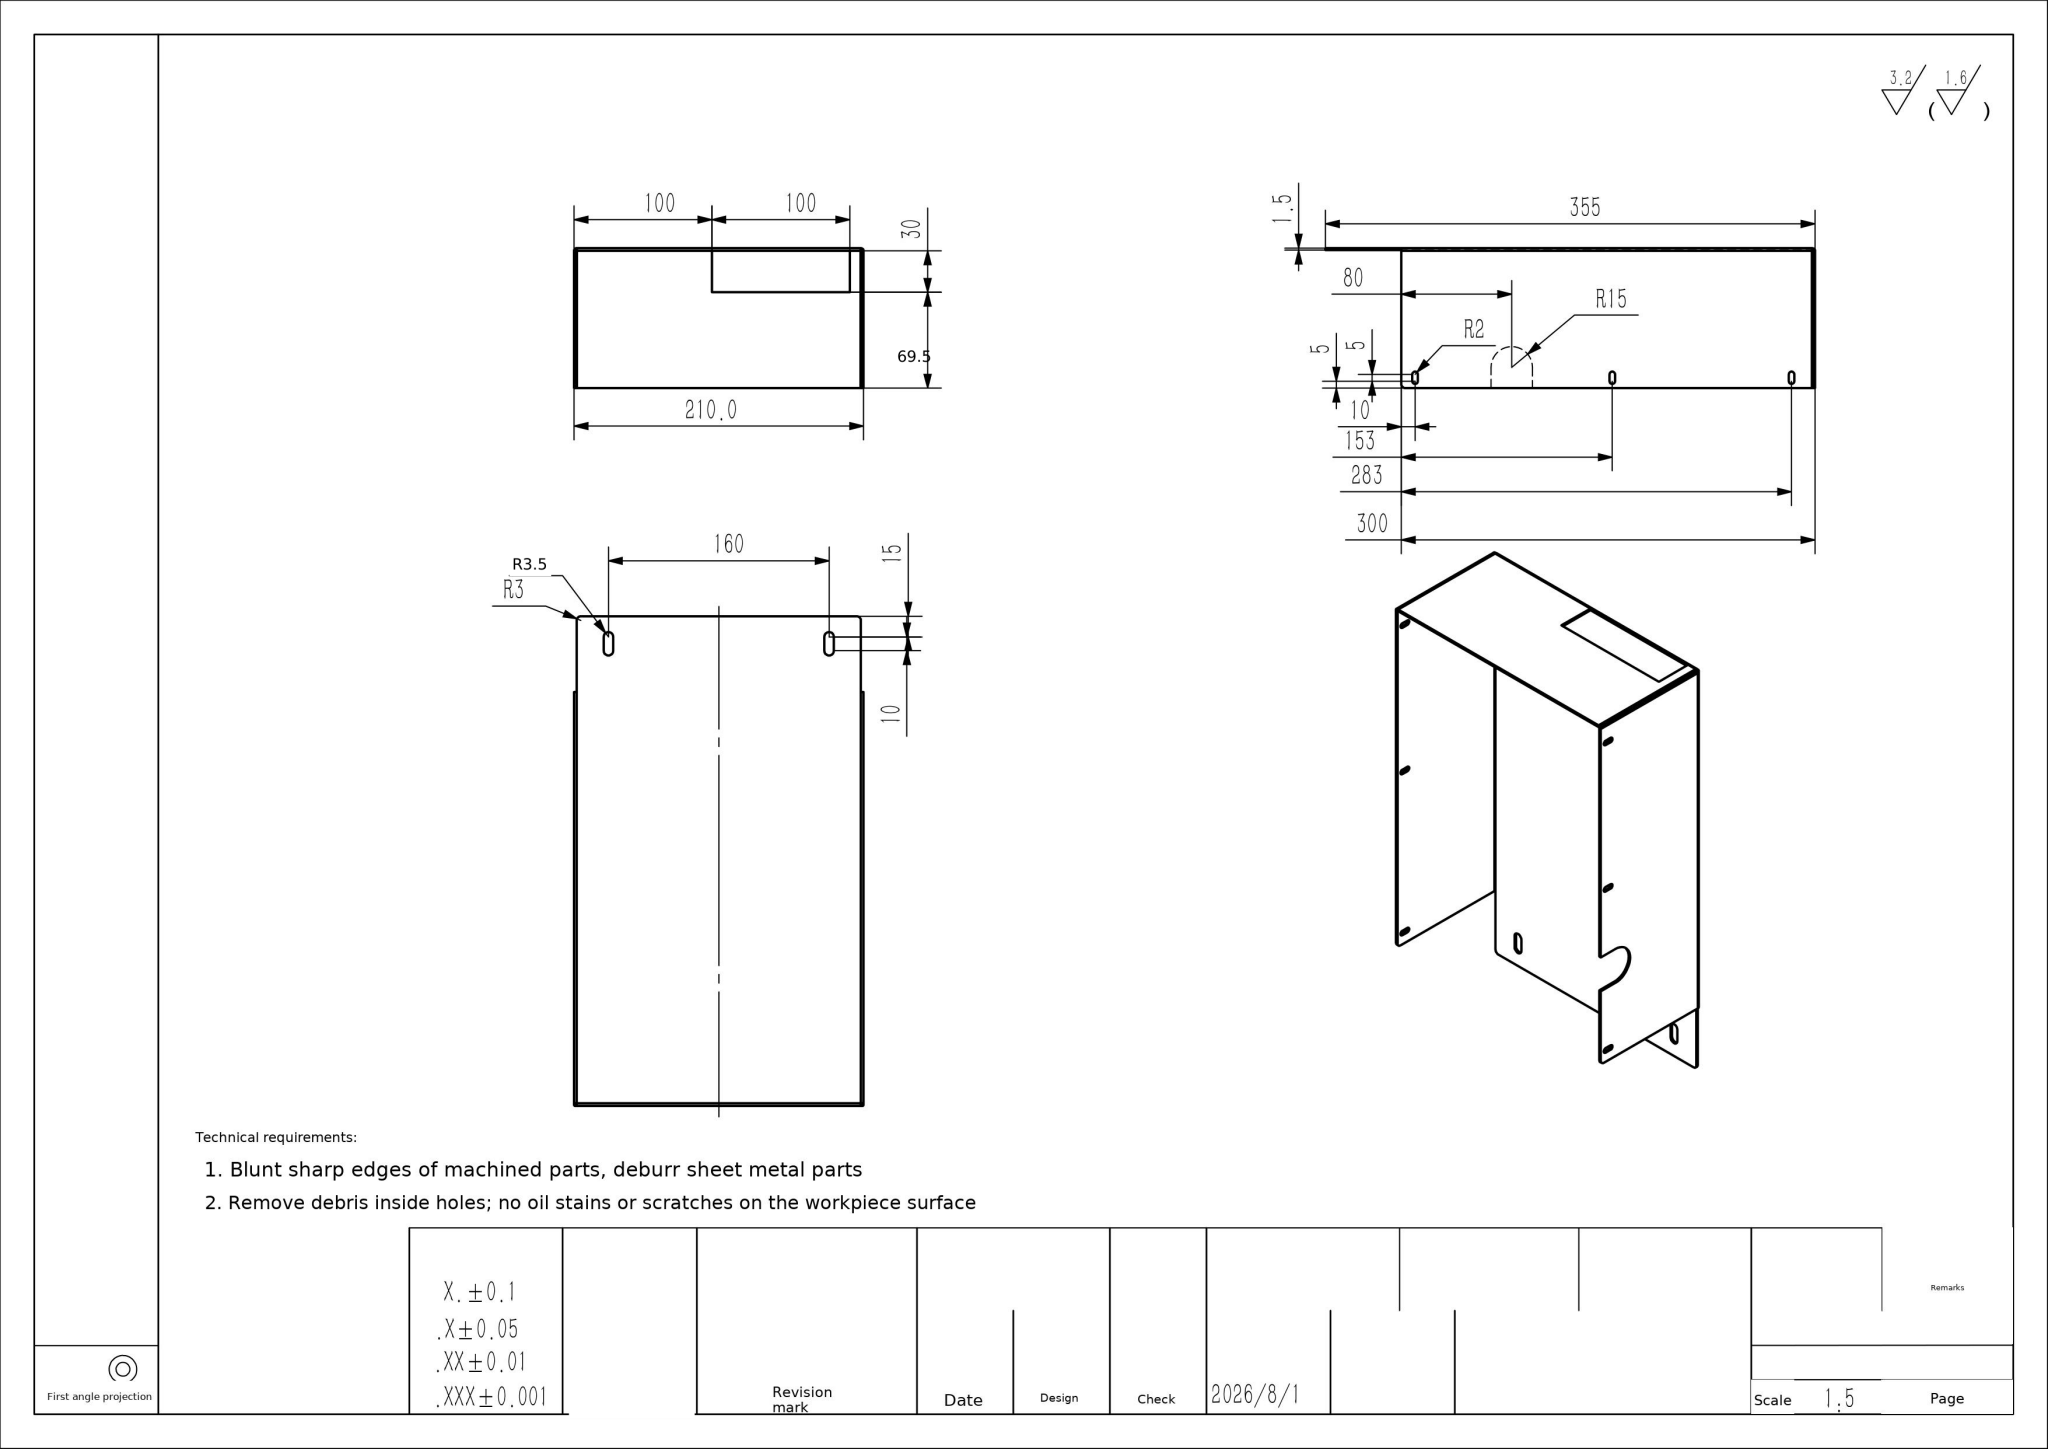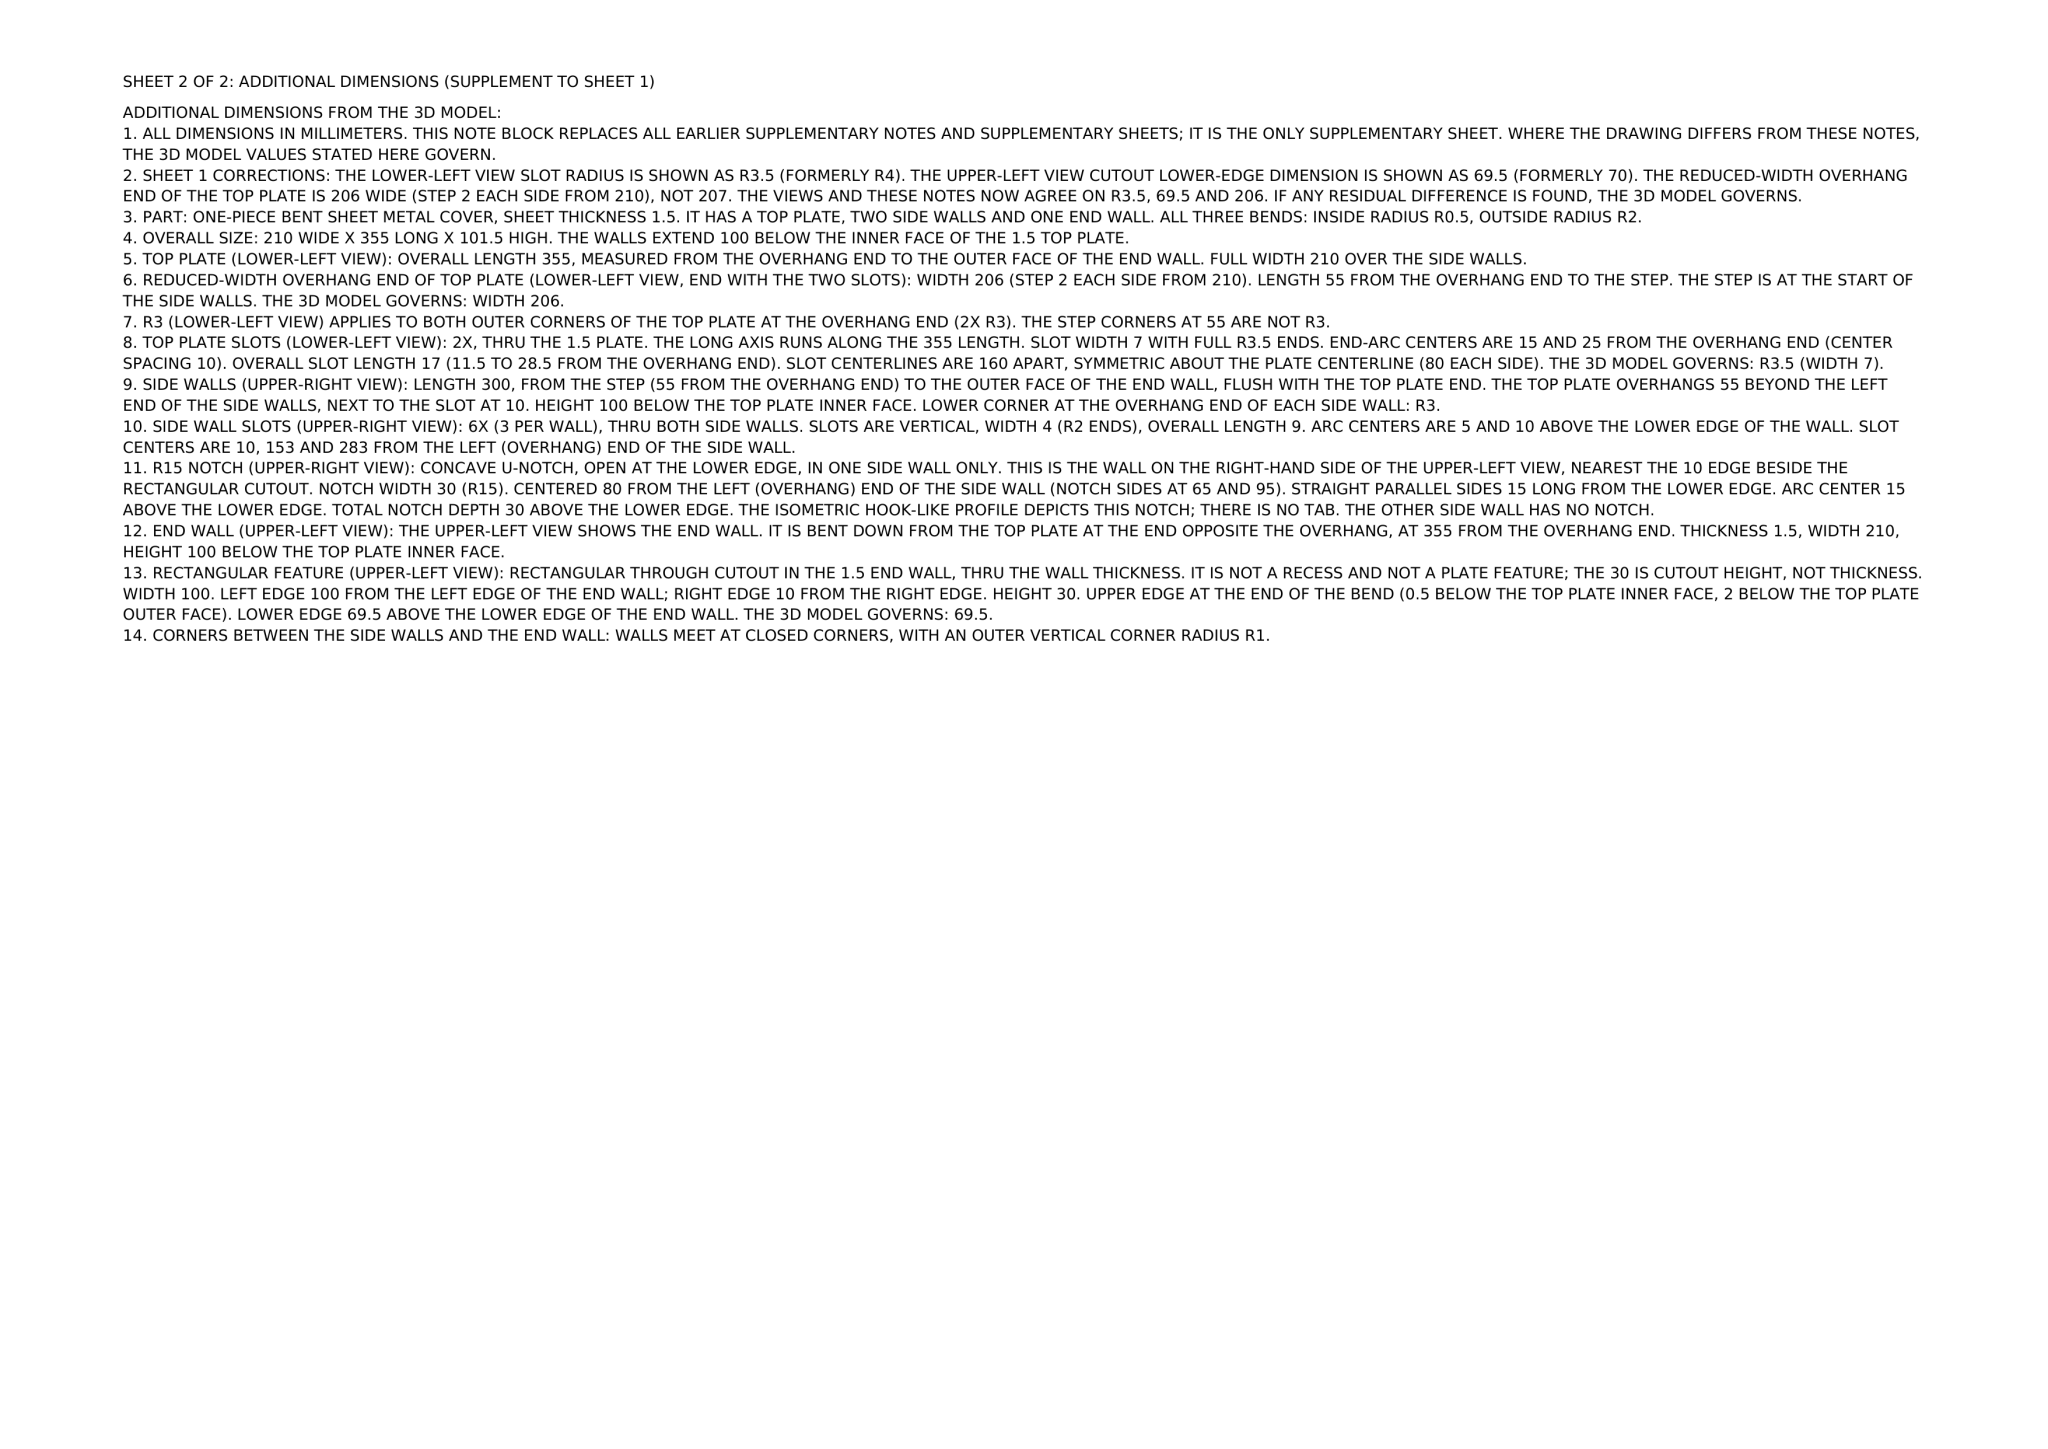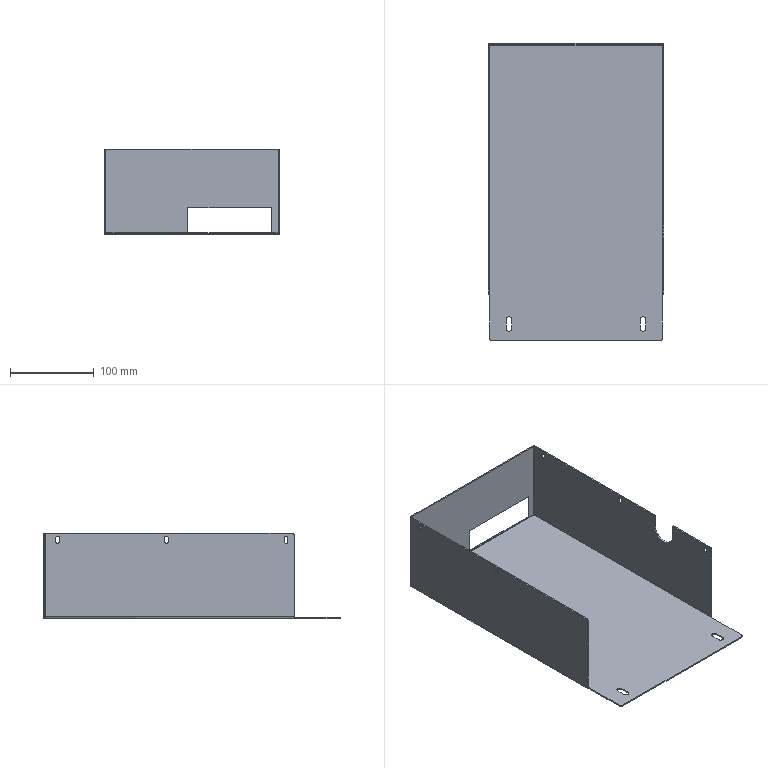Part | NX | mm | 1 solid | 97 faces | box 210 x 355 x 101.5 mm | volume 225516 mm3 | plane 51 | cylinder 36 | spline 10 | commonest cylinder face diameters 4 x21 7 x4 6 x4 1 x3 30 x2 2 x2